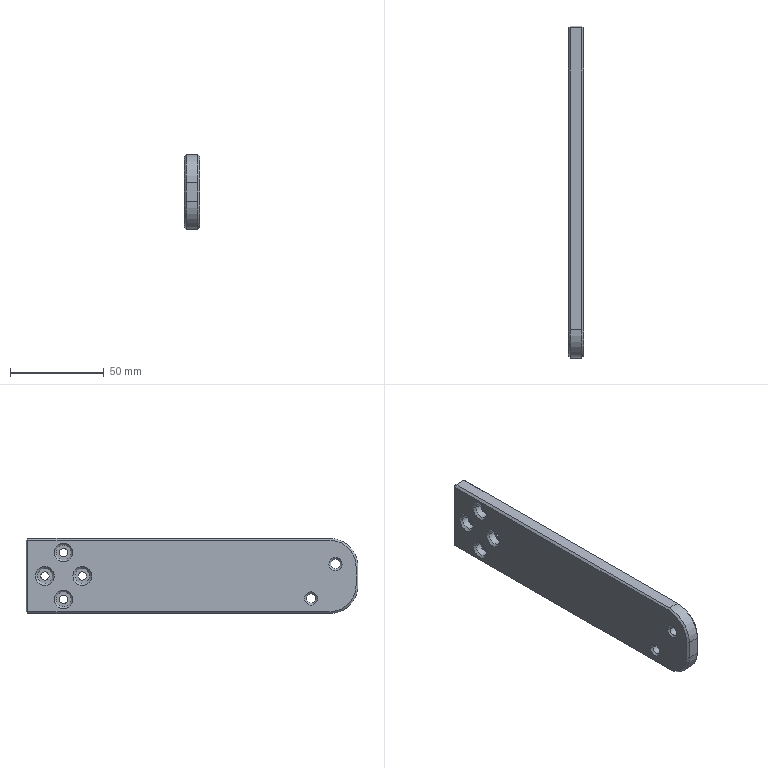Component | SolidWorks | CameraAssembly-1_CameraFixingPlate-1 | 1 solid | 74 faces | box 8 x 177 x 40 mm | volume 53864 mm3 | cone 28 | plane 24 | cylinder 22 | commonest cylinder face diameters 8 x8 4.5 x8 5 x4 30 x2 | material 1060 Alloy
build123d program:
from build123d import *

# Parameters (mm, degrees)
SKETCH1_W                                          = 177
SKETCH1_H                                          = 40
BOSS_EXTRUDE1_DEPTH                                = 8
HOLE_SIZE_ACCORDING_TO_TYPE_OF_HEXAGON_D           = 4.5
HOLE_SIZE_ACCORDING_TO_TYPE_OF_HEXAGON_CBORE_D     = 8
HOLE_SIZE_ACCORDING_TO_TYPE_OF_HEXAGON_CBORE_DEPTH = 4.6
M6_TAPPED_HOLE1_D                                  = 5
FILLET1_R                                          = 15
CHAMFER1_SIZE                                      = 1


with BuildPart() as part:
    # Sketch1 → Boss-Extrude1 (new body)
    with BuildSketch(Plane.XY):
        with Locations((88.5, 0)):
            Rectangle(SKETCH1_W, SKETCH1_H)
    extrude(amount=BOSS_EXTRUDE1_DEPTH)

    # Hole Size _according to_ type of Hexagon (through all)
    with Locations(Plane.XY.offset(8)):
        with Locations((157, -12.5), (157, 12.5), (167, 0), (147, 0)):
            CounterBoreHole(HOLE_SIZE_ACCORDING_TO_TYPE_OF_HEXAGON_D / 2, HOLE_SIZE_ACCORDING_TO_TYPE_OF_HEXAGON_CBORE_D / 2, HOLE_SIZE_ACCORDING_TO_TYPE_OF_HEXAGON_CBORE_DEPTH)

    # M6 Tapped Hole1 (through all)
    with Locations(Plane.XY.offset(8)):
        with Locations((25, 12), (12, -6.364)):
            Hole(M6_TAPPED_HOLE1_D / 2)

    # Fillet1
    fillet1_edges = [part.edges().sort_by_distance(p)[0] for p in [
        (0, 20, 4),
        (0, -20, 4),
    ]]
    fillet(fillet1_edges, radius=FILLET1_R)

    # Chamfer1
    chamfer1_edges = [part.edges().sort_by_distance(p)[0] for p in [
        (177, 0, 8),
        (96, 20, 8),
        (143, 0, 8),
        (149.25, 0, 0),
        (163, 0, 8),
        (169.25, 0, 0),
        (153, 12.5, 8),
        (159.25, 12.5, 0),
        (153, -12.5, 8),
        (159.25, -12.5, 0),
        (96, 20, 0),
        (14.5, -6.364, 8),
        (14.5, -6.364, 0),
        (177, 0, 0),
        (27.5, 12, 8),
        (27.5, 12, 0),
        (96, -20, 0),
        (96, -20, 8),
        (0, 0, 0),
        (4.393, 15.607, 0),
        (4.393, -15.607, 0),
        (0, 0, 8),
        (4.393, 15.607, 8),
        (4.393, -15.607, 8),
        (177, 20, 4),
        (177, -20, 4),
    ]]
    chamfer(chamfer1_edges, length=CHAMFER1_SIZE)


solid = part.part

# Placed as in the assembly
solid = solid.moved(Location((-109.166, 190.264, -287.5), (-90, -90, 0)))